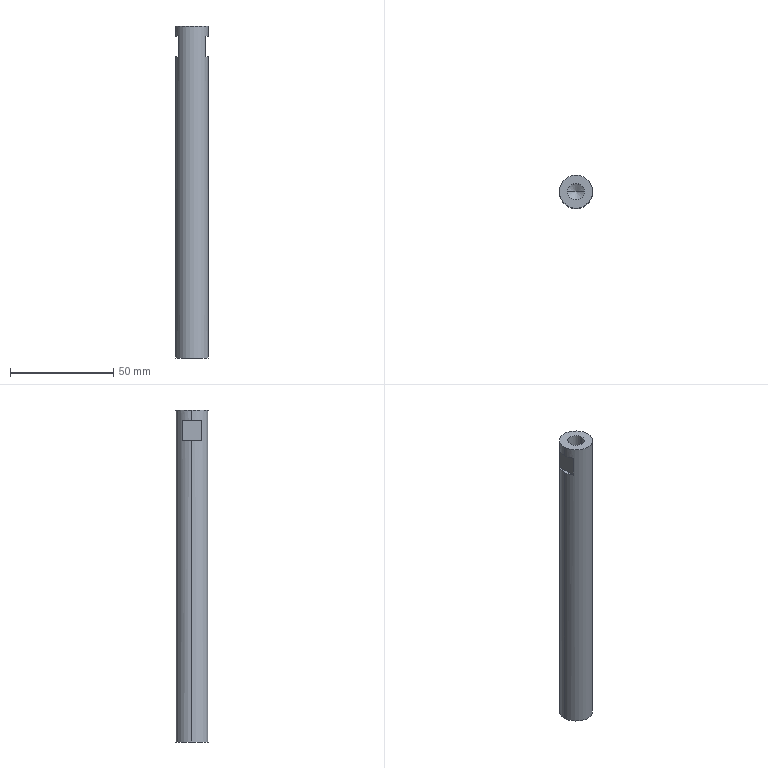Component | SolidWorks | YS01-057LiftingGuideRod-2 | 1 solid | 18 faces | box 16 x 16 x 161 mm | volume 30115 mm3 | plane 8 | cylinder 6 | cone 4 | commonest cylinder face diameters 8 x4 16 x2
build123d program:
from build123d import *

# Parameters (mm, degrees)
SKETCH1_R             = 8
BOSS_EXTRUDE1_DEPTH   = 161
M8_TAPPED_HOLE1_D     = 8
M8_TAPPED_HOLE1_DEPTH = 19.75
M8_TAPPED_HOLE1_TIP   = 2.403
M8_TAPPED_HOLE2_D     = 8
M8_TAPPED_HOLE2_DEPTH = 19.75
M8_TAPPED_HOLE2_TIP   = 2.403
SKETCH6_W             = 13.182
SKETCH6_H             = 34.542
SKETCH6_W_2           = 6.96
SKETCH6_H_2           = 27.136
CUT_EXTRUDE1_DEPTH    = 10


with BuildPart() as part:
    # Sketch1 → Boss-Extrude1 (new body)
    with BuildSketch(Plane.XY):
        with Locations((-70, -20)):
            Circle(SKETCH1_R)
    extrude(amount=BOSS_EXTRUDE1_DEPTH)

    # M8 Tapped Hole1
    with Locations(Plane.XY.offset(161)):
        with Locations((-70, -20)):
            Hole(M8_TAPPED_HOLE1_D / 2, depth=M8_TAPPED_HOLE1_DEPTH)
            with Locations((0, 0, -(M8_TAPPED_HOLE1_DEPTH + M8_TAPPED_HOLE1_TIP / 2))):  # 118° drill point
                Cone(0, M8_TAPPED_HOLE1_D / 2, M8_TAPPED_HOLE1_TIP, mode=Mode.SUBTRACT)

    # M8 Tapped Hole2
    with Locations(Plane(origin=(0, 0, 0), x_dir=(-1, 0, 0), z_dir=(0, 0, -1))):
        with Locations((70, -20)):
            Hole(M8_TAPPED_HOLE2_D / 2, depth=M8_TAPPED_HOLE2_DEPTH)
            with Locations((0, 0, -(M8_TAPPED_HOLE2_DEPTH + M8_TAPPED_HOLE2_TIP / 2))):  # 118° drill point
                Cone(0, M8_TAPPED_HOLE2_D / 2, M8_TAPPED_HOLE2_TIP, mode=Mode.SUBTRACT)

    # Sketch6 → Cut-Extrude1 (cut)
    with BuildSketch(Plane.XY.offset(156)):
        with Locations((-83.091, -25.619)):
            Rectangle(SKETCH6_W, SKETCH6_H)
        with Locations((-60.02, -21.916)):
            Rectangle(SKETCH6_W_2, SKETCH6_H_2)
    extrude(amount=-CUT_EXTRUDE1_DEPTH, mode=Mode.SUBTRACT)


solid = part.part

# Placed as in the assembly
solid = solid.moved(Location((-566.612, -103.873, 2357.4), (0, 0, 0)))
STEP:
#1=COLOUR_RGB('',0.7922,0.8196,0.9333);
#2=FILL_AREA_STYLE_COLOUR('',#1);
#3=FILL_AREA_STYLE('',(#2));
#4=SURFACE_STYLE_FILL_AREA(#3);
#5=SURFACE_SIDE_STYLE('',(#4));
#6=SURFACE_STYLE_USAGE(.BOTH.,#5);
#7=PRESENTATION_STYLE_ASSIGNMENT((#6));
#8=CARTESIAN_POINT('',(-25.221,-4.877,93.589));
#9=VERTEX_POINT('',#8);
#10=CARTESIAN_POINT('',(-24.906,-4.877,93.589));
#11=VERTEX_POINT('',#10);
#12=CARTESIAN_POINT('',(-25.063,-4.877,93.589));
#13=DIRECTION('',(0.,0.,-1.));
#14=DIRECTION('',(1.,0.,0.));
#15=AXIS2_PLACEMENT_3D('',#12,#13,#14);
#16=CIRCLE('',#15,0.1575);
#17=EDGE_CURVE('',#9,#11,#16,.T.);
#18=ORIENTED_EDGE('',*,*,#17,.F.);
#19=CARTESIAN_POINT('',(-25.221,-4.877,92.811));
#20=VERTEX_POINT('',#19);
#21=CARTESIAN_POINT('',(-25.221,-4.877,92.811));
#22=DIRECTION('',(0.,0.,-1.));
#23=VECTOR('',#22,39.37);
#24=LINE('',#21,#23);
#25=EDGE_CURVE('',#9,#20,#24,.T.);
#26=ORIENTED_EDGE('',*,*,#25,.T.);
#27=CARTESIAN_POINT('',(-24.906,-4.877,92.811));
#28=VERTEX_POINT('',#27);
#29=CARTESIAN_POINT('',(-25.063,-4.877,92.811));
#30=DIRECTION('',(0.,0.,-1.));
#31=DIRECTION('',(1.,0.,0.));
#32=AXIS2_PLACEMENT_3D('',#29,#30,#31);
#33=CIRCLE('',#32,0.1575);
#34=EDGE_CURVE('',#20,#28,#33,.T.);
#35=ORIENTED_EDGE('',*,*,#34,.T.);
#36=CARTESIAN_POINT('',(-24.906,-4.877,92.811));
#37=DIRECTION('',(0.,0.,-1.));
#38=VECTOR('',#37,39.37);
#39=LINE('',#36,#38);
#40=EDGE_CURVE('',#11,#28,#39,.T.);
#41=ORIENTED_EDGE('',*,*,#40,.F.);
#42=EDGE_LOOP('',(#18,#26,#35,#41));
#43=FACE_OUTER_BOUND('',#42,.T.);
#44=CARTESIAN_POINT('',(-25.063,-4.877,92.811));
#45=DIRECTION('',(0.,0.,-1.));
#46=DIRECTION('',(1.,0.,0.));
#47=AXIS2_PLACEMENT_3D('',#44,#45,#46);
#48=CYLINDRICAL_SURFACE('',#47,0.1575);
#49=ADVANCED_FACE('',(#43),#48,.F.);
#50=CARTESIAN_POINT('',(-25.063,-4.877,93.683));
#51=VERTEX_POINT('',#50);
#52=CARTESIAN_POINT('',(-24.906,-4.877,93.589));
#53=DIRECTION('',(0.8572,-0.,-0.515));
#54=VECTOR('',#53,39.37);
#55=LINE('',#52,#54);
#56=EDGE_CURVE('',#51,#11,#55,.T.);
#57=ORIENTED_EDGE('',*,*,#56,.F.);
#58=CARTESIAN_POINT('',(-25.221,-4.877,93.589));
#59=DIRECTION('',(-0.8572,-0.,-0.515));
#60=VECTOR('',#59,39.37);
#61=LINE('',#58,#60);
#62=EDGE_CURVE('',#51,#9,#61,.T.);
#63=ORIENTED_EDGE('',*,*,#62,.T.);
#64=ORIENTED_EDGE('',*,*,#17,.T.);
#65=EDGE_LOOP('',(#57,#63,#64));
#66=FACE_OUTER_BOUND('',#65,.T.);
#67=CARTESIAN_POINT('',(-25.063,-4.877,93.589));
#68=DIRECTION('',(0.,0.,-1.));
#69=DIRECTION('',(1.,0.,0.));
#70=AXIS2_PLACEMENT_3D('',#67,#68,#69);
#71=CONICAL_SURFACE('',#70,0.1575,1.03);
#72=ADVANCED_FACE('',(#66),#71,.F.);
#73=CARTESIAN_POINT('',(-24.906,-4.877,98.372));
#74=VERTEX_POINT('',#73);
#75=CARTESIAN_POINT('',(-25.221,-4.877,98.372));
#76=VERTEX_POINT('',#75);
#77=CARTESIAN_POINT('',(-25.063,-4.877,98.372));
#78=DIRECTION('',(0.,0.,1.));
#79=DIRECTION('',(-1.,0.,0.));
#80=AXIS2_PLACEMENT_3D('',#77,#78,#79);
#81=CIRCLE('',#80,0.1575);
#82=EDGE_CURVE('',#74,#76,#81,.T.);
#83=ORIENTED_EDGE('',*,*,#82,.F.);
#84=CARTESIAN_POINT('',(-24.906,-4.877,99.15));
#85=VERTEX_POINT('',#84);
#86=CARTESIAN_POINT('',(-24.906,-4.877,99.15));
#87=DIRECTION('',(0.,0.,1.));
#88=VECTOR('',#87,39.37);
#89=LINE('',#86,#88);
#90=EDGE_CURVE('',#74,#85,#89,.T.);
#91=ORIENTED_EDGE('',*,*,#90,.T.);
#92=CARTESIAN_POINT('',(-25.221,-4.877,99.15));
#93=VERTEX_POINT('',#92);
#94=CARTESIAN_POINT('',(-25.063,-4.877,99.15));
#95=DIRECTION('',(0.,0.,1.));
#96=DIRECTION('',(-1.,0.,0.));
#97=AXIS2_PLACEMENT_3D('',#94,#95,#96);
#98=CIRCLE('',#97,0.1575);
#99=EDGE_CURVE('',#85,#93,#98,.T.);
#100=ORIENTED_EDGE('',*,*,#99,.T.);
#101=CARTESIAN_POINT('',(-25.221,-4.877,99.15));
#102=DIRECTION('',(0.,0.,1.));
#103=VECTOR('',#102,39.37);
#104=LINE('',#101,#103);
#105=EDGE_CURVE('',#76,#93,#104,.T.);
#106=ORIENTED_EDGE('',*,*,#105,.F.);
#107=EDGE_LOOP('',(#83,#91,#100,#106));
#108=FACE_OUTER_BOUND('',#107,.T.);
#109=CARTESIAN_POINT('',(-25.063,-4.877,99.15));
#110=DIRECTION('',(0.,0.,1.));
#111=DIRECTION('',(-1.,0.,0.));
#112=AXIS2_PLACEMENT_3D('',#109,#110,#111);
#113=CYLINDRICAL_SURFACE('',#112,0.1575);
#114=ADVANCED_FACE('',(#108),#113,.F.);
#115=CARTESIAN_POINT('',(-25.063,-4.877,98.277));
#116=VERTEX_POINT('',#115);
#117=CARTESIAN_POINT('',(-25.221,-4.877,98.372));
#118=DIRECTION('',(-0.8572,0.,0.515));
#119=VECTOR('',#118,39.37);
#120=LINE('',#117,#119);
#121=EDGE_CURVE('',#116,#76,#120,.T.);
#122=ORIENTED_EDGE('',*,*,#121,.F.);
#123=CARTESIAN_POINT('',(-24.906,-4.877,98.372));
#124=DIRECTION('',(0.8572,-0.,0.515));
#125=VECTOR('',#124,39.37);
#126=LINE('',#123,#125);
#127=EDGE_CURVE('',#116,#74,#126,.T.);
#128=ORIENTED_EDGE('',*,*,#127,.T.);
#129=ORIENTED_EDGE('',*,*,#82,.T.);
#130=EDGE_LOOP('',(#122,#128,#129));
#131=FACE_OUTER_BOUND('',#130,.T.);
#132=CARTESIAN_POINT('',(-25.063,-4.877,98.372));
#133=DIRECTION('',(0.,0.,1.));
#134=DIRECTION('',(-1.,0.,0.));
#135=AXIS2_PLACEMENT_3D('',#132,#133,#134);
#136=CONICAL_SURFACE('',#135,0.1575,1.03);
#137=ADVANCED_FACE('',(#131),#136,.F.);
#138=CARTESIAN_POINT('',(-25.378,-4.877,99.15));
#139=VERTEX_POINT('',#138);
#140=CARTESIAN_POINT('',(-24.749,-4.877,99.15));
#141=VERTEX_POINT('',#140);
#142=CARTESIAN_POINT('',(-25.063,-4.877,99.15));
#143=DIRECTION('',(0.,0.,1.));
#144=DIRECTION('',(-1.,0.,0.));
#145=AXIS2_PLACEMENT_3D('',#142,#143,#144);
#146=CIRCLE('',#145,0.315);
#147=EDGE_CURVE('',#139,#141,#146,.T.);
#148=ORIENTED_EDGE('',*,*,#147,.F.);
#149=CARTESIAN_POINT('',(-25.378,-4.877,98.953));
#150=VERTEX_POINT('',#149);
#151=CARTESIAN_POINT('',(-25.378,-4.877,99.15));
#152=DIRECTION('',(0.,0.,-1.));
#153=VECTOR('',#152,39.37);
#154=LINE('',#151,#153);
#155=EDGE_CURVE('',#139,#150,#154,.T.);
#156=ORIENTED_EDGE('',*,*,#155,.T.);
#157=CARTESIAN_POINT('',(-25.319,-5.061,98.953));
#158=VERTEX_POINT('',#157);
#159=CARTESIAN_POINT('',(-25.063,-4.877,98.953));
#160=DIRECTION('',(0.,0.,1.));
#161=DIRECTION('',(-1.,0.,0.));
#162=AXIS2_PLACEMENT_3D('',#159,#160,#161);
#163=CIRCLE('',#162,0.315);
#164=EDGE_CURVE('',#150,#158,#163,.T.);
#165=ORIENTED_EDGE('',*,*,#164,.T.);
#166=CARTESIAN_POINT('',(-25.319,-5.061,98.559));
#167=VERTEX_POINT('',#166);
#168=CARTESIAN_POINT('',(-25.319,-5.061,99.15));
#169=DIRECTION('',(0.,0.,1.));
#170=VECTOR('',#169,39.37);
#171=LINE('',#168,#170);
#172=EDGE_CURVE('',#167,#158,#171,.T.);
#173=ORIENTED_EDGE('',*,*,#172,.F.);
#174=CARTESIAN_POINT('',(-25.378,-4.877,98.559));
#175=VERTEX_POINT('',#174);
#176=CARTESIAN_POINT('',(-25.063,-4.877,98.559));
#177=DIRECTION('',(0.,0.,1.));
#178=DIRECTION('',(-1.,0.,0.));
#179=AXIS2_PLACEMENT_3D('',#176,#177,#178);
#180=CIRCLE('',#179,0.315);
#181=EDGE_CURVE('',#175,#167,#180,.T.);
#182=ORIENTED_EDGE('',*,*,#181,.F.);
#183=CARTESIAN_POINT('',(-25.378,-4.877,92.811));
#184=VERTEX_POINT('',#183);
#185=CARTESIAN_POINT('',(-25.378,-4.877,99.15));
#186=DIRECTION('',(0.,0.,-1.));
#187=VECTOR('',#186,39.37);
#188=LINE('',#185,#187);
#189=EDGE_CURVE('',#175,#184,#188,.T.);
#190=ORIENTED_EDGE('',*,*,#189,.T.);
#191=CARTESIAN_POINT('',(-24.749,-4.877,92.811));
#192=VERTEX_POINT('',#191);
#193=CARTESIAN_POINT('',(-25.063,-4.877,92.811));
#194=DIRECTION('',(0.,0.,1.));
#195=DIRECTION('',(-1.,0.,0.));
#196=AXIS2_PLACEMENT_3D('',#193,#194,#195);
#197=CIRCLE('',#196,0.315);
#198=EDGE_CURVE('',#184,#192,#197,.T.);
#199=ORIENTED_EDGE('',*,*,#198,.T.);
#200=CARTESIAN_POINT('',(-24.749,-4.877,98.559));
#201=VERTEX_POINT('',#200);
#202=CARTESIAN_POINT('',(-24.749,-4.877,99.15));
#203=DIRECTION('',(0.,0.,-1.));
#204=VECTOR('',#203,39.37);
#205=LINE('',#202,#204);
#206=EDGE_CURVE('',#201,#192,#205,.T.);
#207=ORIENTED_EDGE('',*,*,#206,.F.);
#208=CARTESIAN_POINT('',(-24.808,-5.061,98.559));
#209=VERTEX_POINT('',#208);
#210=CARTESIAN_POINT('',(-25.063,-4.877,98.559));
#211=DIRECTION('',(0.,0.,-1.));
#212=DIRECTION('',(1.,0.,0.));
#213=AXIS2_PLACEMENT_3D('',#210,#211,#212);
#214=CIRCLE('',#213,0.315);
#215=EDGE_CURVE('',#201,#209,#214,.T.);
#216=ORIENTED_EDGE('',*,*,#215,.T.);
#217=CARTESIAN_POINT('',(-24.808,-5.061,98.953));
#218=VERTEX_POINT('',#217);
#219=CARTESIAN_POINT('',(-24.808,-5.061,99.15));
#220=DIRECTION('',(0.,0.,1.));
#221=VECTOR('',#220,39.37);
#222=LINE('',#219,#221);
#223=EDGE_CURVE('',#209,#218,#222,.T.);
#224=ORIENTED_EDGE('',*,*,#223,.T.);
#225=CARTESIAN_POINT('',(-24.749,-4.877,98.953));
#226=VERTEX_POINT('',#225);
#227=CARTESIAN_POINT('',(-25.063,-4.877,98.953));
#228=DIRECTION('',(0.,0.,-1.));
#229=DIRECTION('',(1.,0.,0.));
#230=AXIS2_PLACEMENT_3D('',#227,#228,#229);
#231=CIRCLE('',#230,0.315);
#232=EDGE_CURVE('',#226,#218,#231,.T.);
#233=ORIENTED_EDGE('',*,*,#232,.F.);
#234=CARTESIAN_POINT('',(-24.749,-4.877,99.15));
#235=DIRECTION('',(0.,0.,-1.));
#236=VECTOR('',#235,39.37);
#237=LINE('',#234,#236);
#238=EDGE_CURVE('',#141,#226,#237,.T.);
#239=ORIENTED_EDGE('',*,*,#238,.F.);
#240=EDGE_LOOP('',(#148,#156,#165,#173,#182,#190,#199,#207,#216,#224,#233,#239));
#241=FACE_OUTER_BOUND('',#240,.T.);
#242=CARTESIAN_POINT('',(-25.063,-4.877,99.15));
#243=DIRECTION('',(0.,0.,-1.));
#244=DIRECTION('',(1.,0.,0.));
#245=AXIS2_PLACEMENT_3D('',#242,#243,#244);
#246=CYLINDRICAL_SURFACE('',#245,0.315);
#247=ADVANCED_FACE('',(#241),#246,.T.);
#248=ORIENTED_EDGE('',*,*,#155,.F.);
#249=CARTESIAN_POINT('',(-25.063,-4.877,99.15));
#250=DIRECTION('',(0.,0.,1.));
#251=DIRECTION('',(-1.,0.,0.));
#252=AXIS2_PLACEMENT_3D('',#249,#250,#251);
#253=CIRCLE('',#252,0.315);
#254=EDGE_CURVE('',#141,#139,#253,.T.);
#255=ORIENTED_EDGE('',*,*,#254,.F.);
#256=ORIENTED_EDGE('',*,*,#238,.T.);
#257=CARTESIAN_POINT('',(-24.808,-4.693,98.953));
#258=VERTEX_POINT('',#257);
#259=CARTESIAN_POINT('',(-25.063,-4.877,98.953));
#260=DIRECTION('',(0.,0.,-1.));
#261=DIRECTION('',(1.,0.,0.));
#262=AXIS2_PLACEMENT_3D('',#259,#260,#261);
#263=CIRCLE('',#262,0.315);
#264=EDGE_CURVE('',#258,#226,#263,.T.);
#265=ORIENTED_EDGE('',*,*,#264,.F.);
#266=CARTESIAN_POINT('',(-24.808,-4.693,98.559));
#267=VERTEX_POINT('',#266);
#268=CARTESIAN_POINT('',(-24.808,-4.693,99.15));
#269=DIRECTION('',(0.,0.,-1.));
#270=VECTOR('',#269,39.37);
#271=LINE('',#268,#270);
#272=EDGE_CURVE('',#258,#267,#271,.T.);
#273=ORIENTED_EDGE('',*,*,#272,.T.);
#274=CARTESIAN_POINT('',(-25.063,-4.877,98.559));
#275=DIRECTION('',(0.,0.,-1.));
#276=DIRECTION('',(1.,0.,0.));
#277=AXIS2_PLACEMENT_3D('',#274,#275,#276);
#278=CIRCLE('',#277,0.315);
#279=EDGE_CURVE('',#267,#201,#278,.T.);
#280=ORIENTED_EDGE('',*,*,#279,.T.);
#281=ORIENTED_EDGE('',*,*,#206,.T.);
#282=CARTESIAN_POINT('',(-25.063,-4.877,92.811));
#283=DIRECTION('',(0.,0.,1.));
#284=DIRECTION('',(-1.,0.,0.));
#285=AXIS2_PLACEMENT_3D('',#282,#283,#284);
#286=CIRCLE('',#285,0.315);
#287=EDGE_CURVE('',#192,#184,#286,.T.);
#288=ORIENTED_EDGE('',*,*,#287,.T.);
#289=ORIENTED_EDGE('',*,*,#189,.F.);
#290=CARTESIAN_POINT('',(-25.319,-4.693,98.559));
#291=VERTEX_POINT('',#290);
#292=CARTESIAN_POINT('',(-25.063,-4.877,98.559));
#293=DIRECTION('',(0.,0.,1.));
#294=DIRECTION('',(-1.,0.,0.));
#295=AXIS2_PLACEMENT_3D('',#292,#293,#294);
#296=CIRCLE('',#295,0.315);
#297=EDGE_CURVE('',#291,#175,#296,.T.);
#298=ORIENTED_EDGE('',*,*,#297,.F.);
#299=CARTESIAN_POINT('',(-25.319,-4.693,98.953));
#300=VERTEX_POINT('',#299);
#301=CARTESIAN_POINT('',(-25.319,-4.693,99.15));
#302=DIRECTION('',(0.,0.,-1.));
#303=VECTOR('',#302,39.37);
#304=LINE('',#301,#303);
#305=EDGE_CURVE('',#300,#291,#304,.T.);
#306=ORIENTED_EDGE('',*,*,#305,.F.);
#307=CARTESIAN_POINT('',(-25.063,-4.877,98.953));
#308=DIRECTION('',(0.,0.,1.));
#309=DIRECTION('',(-1.,0.,0.));
#310=AXIS2_PLACEMENT_3D('',#307,#308,#309);
#311=CIRCLE('',#310,0.315);
#312=EDGE_CURVE('',#300,#150,#311,.T.);
#313=ORIENTED_EDGE('',*,*,#312,.T.);
#314=EDGE_LOOP('',(#248,#255,#256,#265,#273,#280,#281,#288,#289,#298,#306,#313));
#315=FACE_OUTER_BOUND('',#314,.T.);
#316=CARTESIAN_POINT('',(-25.063,-4.877,99.15));
#317=DIRECTION('',(0.,0.,-1.));
#318=DIRECTION('',(1.,0.,0.));
#319=AXIS2_PLACEMENT_3D('',#316,#317,#318);
#320=CYLINDRICAL_SURFACE('',#319,0.315);
#321=ADVANCED_FACE('',(#315),#320,.T.);
#322=CARTESIAN_POINT('',(-25.063,-4.877,99.15));
#323=DIRECTION('',(0.,0.,1.));
#324=DIRECTION('',(-1.,0.,0.));
#325=AXIS2_PLACEMENT_3D('',#322,#323,#324);
#326=CIRCLE('',#325,0.1575);
#327=EDGE_CURVE('',#93,#85,#326,.T.);
#328=ORIENTED_EDGE('',*,*,#327,.F.);
#329=ORIENTED_EDGE('',*,*,#99,.F.);
#330=EDGE_LOOP('',(#328,#329));
#331=FACE_BOUND('',#330,.T.);
#332=ORIENTED_EDGE('',*,*,#254,.T.);
#333=ORIENTED_EDGE('',*,*,#147,.T.);
#334=EDGE_LOOP('',(#332,#333));
#335=FACE_OUTER_BOUND('',#334,.T.);
#336=CARTESIAN_POINT('',(-25.063,-4.877,99.15));
#337=DIRECTION('',(0.,0.,1.));
#338=DIRECTION('',(-1.,0.,0.));
#339=AXIS2_PLACEMENT_3D('',#336,#337,#338);
#340=PLANE('',#339);
#341=ADVANCED_FACE('',(#331,#335),#340,.T.);
#342=CARTESIAN_POINT('',(-25.063,-4.877,92.811));
#343=DIRECTION('',(0.,0.,-1.));
#344=DIRECTION('',(1.,0.,0.));
#345=AXIS2_PLACEMENT_3D('',#342,#343,#344);
#346=CIRCLE('',#345,0.1575);
#347=EDGE_CURVE('',#28,#20,#346,.T.);
#348=ORIENTED_EDGE('',*,*,#347,.F.);
#349=ORIENTED_EDGE('',*,*,#34,.F.);
#350=EDGE_LOOP('',(#348,#349));
#351=FACE_BOUND('',#350,.T.);
#352=ORIENTED_EDGE('',*,*,#287,.F.);
#353=ORIENTED_EDGE('',*,*,#198,.F.);
#354=EDGE_LOOP('',(#352,#353));
#355=FACE_OUTER_BOUND('',#354,.T.);
#356=CARTESIAN_POINT('',(-25.063,-4.877,92.811));
#357=DIRECTION('',(0.,0.,1.));
#358=DIRECTION('',(-1.,0.,0.));
#359=AXIS2_PLACEMENT_3D('',#356,#357,#358);
#360=PLANE('',#359);
#361=ADVANCED_FACE('',(#351,#355),#360,.F.);
#362=ORIENTED_EDGE('',*,*,#127,.F.);
#363=ORIENTED_EDGE('',*,*,#121,.T.);
#364=CARTESIAN_POINT('',(-25.063,-4.877,98.372));
#365=DIRECTION('',(0.,0.,1.));
#366=DIRECTION('',(-1.,0.,0.));
#367=AXIS2_PLACEMENT_3D('',#364,#365,#366);
#368=CIRCLE('',#367,0.1575);
#369=EDGE_CURVE('',#76,#74,#368,.T.);
#370=ORIENTED_EDGE('',*,*,#369,.T.);
#371=EDGE_LOOP('',(#362,#363,#370));
#372=FACE_OUTER_BOUND('',#371,.T.);
#373=CARTESIAN_POINT('',(-25.063,-4.877,98.372));
#374=DIRECTION('',(0.,0.,1.));
#375=DIRECTION('',(-1.,0.,0.));
#376=AXIS2_PLACEMENT_3D('',#373,#374,#375);
#377=CONICAL_SURFACE('',#376,0.1575,1.03);
#378=ADVANCED_FACE('',(#372),#377,.F.);
#379=ORIENTED_EDGE('',*,*,#90,.F.);
#380=ORIENTED_EDGE('',*,*,#369,.F.);
#381=ORIENTED_EDGE('',*,*,#105,.T.);
#382=ORIENTED_EDGE('',*,*,#327,.T.);
#383=EDGE_LOOP('',(#379,#380,#381,#382));
#384=FACE_OUTER_BOUND('',#383,.T.);
#385=CARTESIAN_POINT('',(-25.063,-4.877,99.15));
#386=DIRECTION('',(0.,0.,1.));
#387=DIRECTION('',(-1.,0.,0.));
#388=AXIS2_PLACEMENT_3D('',#385,#386,#387);
#389=CYLINDRICAL_SURFACE('',#388,0.1575);
#390=ADVANCED_FACE('',(#384),#389,.F.);
#391=ORIENTED_EDGE('',*,*,#62,.F.);
#392=ORIENTED_EDGE('',*,*,#56,.T.);
#393=CARTESIAN_POINT('',(-25.063,-4.877,93.589));
#394=DIRECTION('',(0.,0.,-1.));
#395=DIRECTION('',(1.,0.,0.));
#396=AXIS2_PLACEMENT_3D('',#393,#394,#395);
#397=CIRCLE('',#396,0.1575);
#398=EDGE_CURVE('',#11,#9,#397,.T.);
#399=ORIENTED_EDGE('',*,*,#398,.T.);
#400=EDGE_LOOP('',(#391,#392,#399));
#401=FACE_OUTER_BOUND('',#400,.T.);
#402=CARTESIAN_POINT('',(-25.063,-4.877,93.589));
#403=DIRECTION('',(0.,0.,-1.));
#404=DIRECTION('',(1.,0.,0.));
#405=AXIS2_PLACEMENT_3D('',#402,#403,#404);
#406=CONICAL_SURFACE('',#405,0.1575,1.03);
#407=ADVANCED_FACE('',(#401),#406,.F.);
#408=ORIENTED_EDGE('',*,*,#25,.F.);
#409=ORIENTED_EDGE('',*,*,#398,.F.);
#410=ORIENTED_EDGE('',*,*,#40,.T.);
#411=ORIENTED_EDGE('',*,*,#347,.T.);
#412=EDGE_LOOP('',(#408,#409,#410,#411));
#413=FACE_OUTER_BOUND('',#412,.T.);
#414=CARTESIAN_POINT('',(-25.063,-4.877,92.811));
#415=DIRECTION('',(0.,0.,-1.));
#416=DIRECTION('',(1.,0.,0.));
#417=AXIS2_PLACEMENT_3D('',#414,#415,#416);
#418=CYLINDRICAL_SURFACE('',#417,0.1575);
#419=ADVANCED_FACE('',(#413),#418,.F.);
#420=CARTESIAN_POINT('',(-24.808,-3.976,98.953));
#421=DIRECTION('',(-0.,-1.,0.));
#422=VECTOR('',#421,39.37);
#423=LINE('',#420,#422);
#424=EDGE_CURVE('',#258,#218,#423,.T.);
#425=ORIENTED_EDGE('',*,*,#424,.T.);
#426=ORIENTED_EDGE('',*,*,#223,.F.);
#427=CARTESIAN_POINT('',(-24.808,-3.976,98.559));
#428=DIRECTION('',(-0.,-1.,0.));
#429=VECTOR('',#428,39.37);
#430=LINE('',#427,#429);
#431=EDGE_CURVE('',#267,#209,#430,.T.);
#432=ORIENTED_EDGE('',*,*,#431,.F.);
#433=ORIENTED_EDGE('',*,*,#272,.F.);
#434=EDGE_LOOP('',(#425,#426,#432,#433));
#435=FACE_OUTER_BOUND('',#434,.T.);
#436=CARTESIAN_POINT('',(-24.808,-3.976,98.559));
#437=DIRECTION('',(-1.,0.,0.));
#438=DIRECTION('',(0.,0.,-1.));
#439=AXIS2_PLACEMENT_3D('',#436,#437,#438);
#440=PLANE('',#439);
#441=ADVANCED_FACE('',(#435),#440,.F.);
#442=ORIENTED_EDGE('',*,*,#431,.T.);
#443=ORIENTED_EDGE('',*,*,#215,.F.);
#444=ORIENTED_EDGE('',*,*,#279,.F.);
#445=EDGE_LOOP('',(#442,#443,#444));
#446=FACE_OUTER_BOUND('',#445,.T.);
#447=CARTESIAN_POINT('',(-27.819,-5.664,98.559));
#448=DIRECTION('',(0.,0.,-1.));
#449=DIRECTION('',(1.,-0.,0.));
#450=AXIS2_PLACEMENT_3D('',#447,#448,#449);
#451=PLANE('',#450);
#452=ADVANCED_FACE('',(#446),#451,.F.);
#453=ORIENTED_EDGE('',*,*,#264,.T.);
#454=ORIENTED_EDGE('',*,*,#232,.T.);
#455=ORIENTED_EDGE('',*,*,#424,.F.);
#456=EDGE_LOOP('',(#453,#454,#455));
#457=FACE_OUTER_BOUND('',#456,.T.);
#458=CARTESIAN_POINT('',(-27.819,-5.664,98.953));
#459=DIRECTION('',(0.,0.,-1.));
#460=DIRECTION('',(1.,-0.,0.));
#461=AXIS2_PLACEMENT_3D('',#458,#459,#460);
#462=PLANE('',#461);
#463=ADVANCED_FACE('',(#457),#462,.T.);
#464=ORIENTED_EDGE('',*,*,#305,.T.);
#465=CARTESIAN_POINT('',(-25.319,-4.267,98.559));
#466=DIRECTION('',(-0.,-1.,0.));
#467=VECTOR('',#466,39.37);
#468=LINE('',#465,#467);
#469=EDGE_CURVE('',#291,#167,#468,.T.);
#470=ORIENTED_EDGE('',*,*,#469,.T.);
#471=ORIENTED_EDGE('',*,*,#172,.T.);
#472=CARTESIAN_POINT('',(-25.319,-4.267,98.953));
#473=DIRECTION('',(-0.,-1.,0.));
#474=VECTOR('',#473,39.37);
#475=LINE('',#472,#474);
#476=EDGE_CURVE('',#300,#158,#475,.T.);
#477=ORIENTED_EDGE('',*,*,#476,.F.);
#478=EDGE_LOOP('',(#464,#470,#471,#477));
#479=FACE_OUTER_BOUND('',#478,.T.);
#480=CARTESIAN_POINT('',(-25.319,-4.267,98.559));
#481=DIRECTION('',(-1.,0.,0.));
#482=DIRECTION('',(0.,0.,-1.));
#483=AXIS2_PLACEMENT_3D('',#480,#481,#482);
#484=PLANE('',#483);
#485=ADVANCED_FACE('',(#479),#484,.T.);
#486=ORIENTED_EDGE('',*,*,#297,.T.);
#487=ORIENTED_EDGE('',*,*,#181,.T.);
#488=ORIENTED_EDGE('',*,*,#469,.F.);
#489=EDGE_LOOP('',(#486,#487,#488));
#490=FACE_OUTER_BOUND('',#489,.T.);
#491=CARTESIAN_POINT('',(-27.819,-5.664,98.559));
#492=DIRECTION('',(0.,0.,1.));
#493=DIRECTION('',(-1.,0.,0.));
#494=AXIS2_PLACEMENT_3D('',#491,#492,#493);
#495=PLANE('',#494);
#496=ADVANCED_FACE('',(#490),#495,.T.);
#497=ORIENTED_EDGE('',*,*,#476,.T.);
#498=ORIENTED_EDGE('',*,*,#164,.F.);
#499=ORIENTED_EDGE('',*,*,#312,.F.);
#500=EDGE_LOOP('',(#497,#498,#499));
#501=FACE_OUTER_BOUND('',#500,.T.);
#502=CARTESIAN_POINT('',(-27.819,-5.664,98.953));
#503=DIRECTION('',(0.,0.,1.));
#504=DIRECTION('',(-1.,0.,0.));
#505=AXIS2_PLACEMENT_3D('',#502,#503,#504);
#506=PLANE('',#505);
#507=ADVANCED_FACE('',(#501),#506,.F.);
#508=CLOSED_SHELL('',(#49,#72,#114,#137,#247,#321,#341,#361,#378,#390,#407,#419,#441,#452,#463,#485,#496,#507));
#509=MANIFOLD_SOLID_BREP('',#508);
#510=STYLED_ITEM('',(#7),#509);
#511=(LENGTH_UNIT()NAMED_UNIT(*)SI_UNIT($,.METRE.));
#512=LENGTH_MEASURE_WITH_UNIT(LENGTH_MEASURE(0.0254),#511);
#513=DIMENSIONAL_EXPONENTS(1.,0.,0.,0.,0.,0.,0.);
#514=(CONVERSION_BASED_UNIT('',#512)LENGTH_UNIT()NAMED_UNIT(#513));
#515=UNCERTAINTY_MEASURE_WITH_UNIT(LENGTH_MEASURE(0.00001),#514,'','');
#516=(NAMED_UNIT(*)PLANE_ANGLE_UNIT()SI_UNIT($,.RADIAN.));
#517=(NAMED_UNIT(*)SI_UNIT($,.STERADIAN.)SOLID_ANGLE_UNIT());
#518=(GEOMETRIC_REPRESENTATION_CONTEXT(3)GLOBAL_UNCERTAINTY_ASSIGNED_CONTEXT((#515))GLOBAL_UNIT_ASSIGNED_CONTEXT((#514,#516,#517))REPRESENTATION_CONTEXT('',''));
#519=MECHANICAL_DESIGN_GEOMETRIC_PRESENTATION_REPRESENTATION('',(#510),#518);
#520=PRESENTATION_LAYER_ASSIGNMENT('','',(#510));
#521=CARTESIAN_POINT('',(0.,0.,0.));
#522=DIRECTION('',(0.,0.,1.));
#523=DIRECTION('',(1.,0.,0.));
#524=AXIS2_PLACEMENT_3D('',#521,#522,#523);
#525=(LENGTH_UNIT()NAMED_UNIT(*)SI_UNIT($,.METRE.));
#526=LENGTH_MEASURE_WITH_UNIT(LENGTH_MEASURE(0.0254),#525);
#527=DIMENSIONAL_EXPONENTS(1.,0.,0.,0.,0.,0.,0.);
#528=(CONVERSION_BASED_UNIT('',#526)LENGTH_UNIT()NAMED_UNIT(#527));
#529=UNCERTAINTY_MEASURE_WITH_UNIT(LENGTH_MEASURE(0.00001),#528,'','');
#530=(NAMED_UNIT(*)PLANE_ANGLE_UNIT()SI_UNIT($,.RADIAN.));
#531=(NAMED_UNIT(*)SI_UNIT($,.STERADIAN.)SOLID_ANGLE_UNIT());
#532=(GEOMETRIC_REPRESENTATION_CONTEXT(3)GLOBAL_UNCERTAINTY_ASSIGNED_CONTEXT((#529))GLOBAL_UNIT_ASSIGNED_CONTEXT((#528,#530,#531))REPRESENTATION_CONTEXT('',''));
#533=ADVANCED_BREP_SHAPE_REPRESENTATION('',(#509,#524),#532);